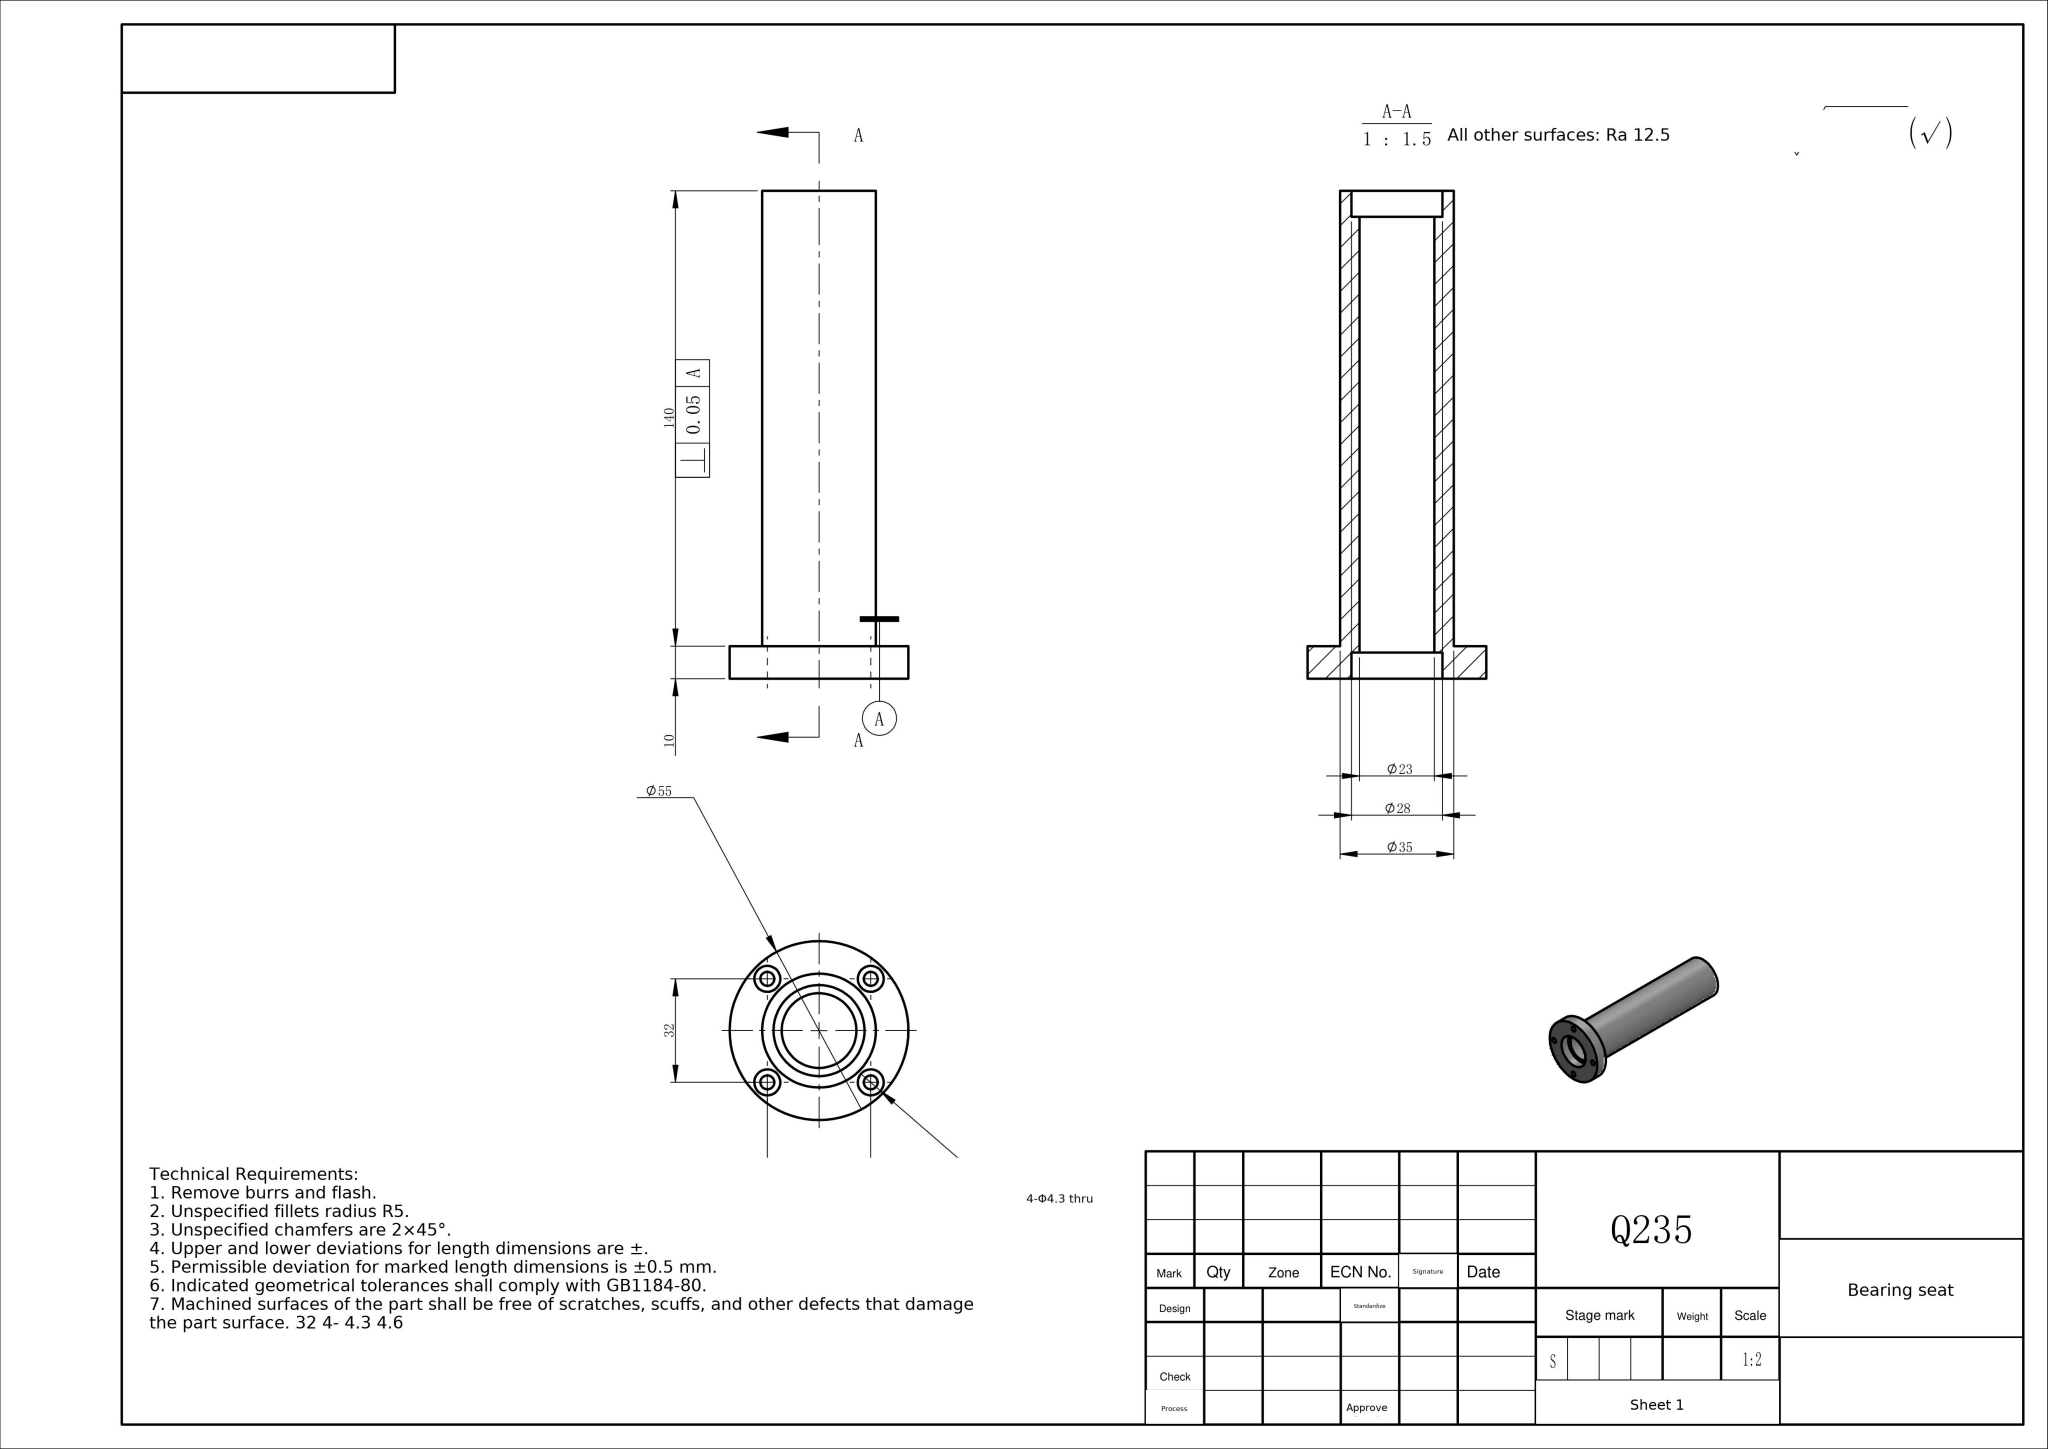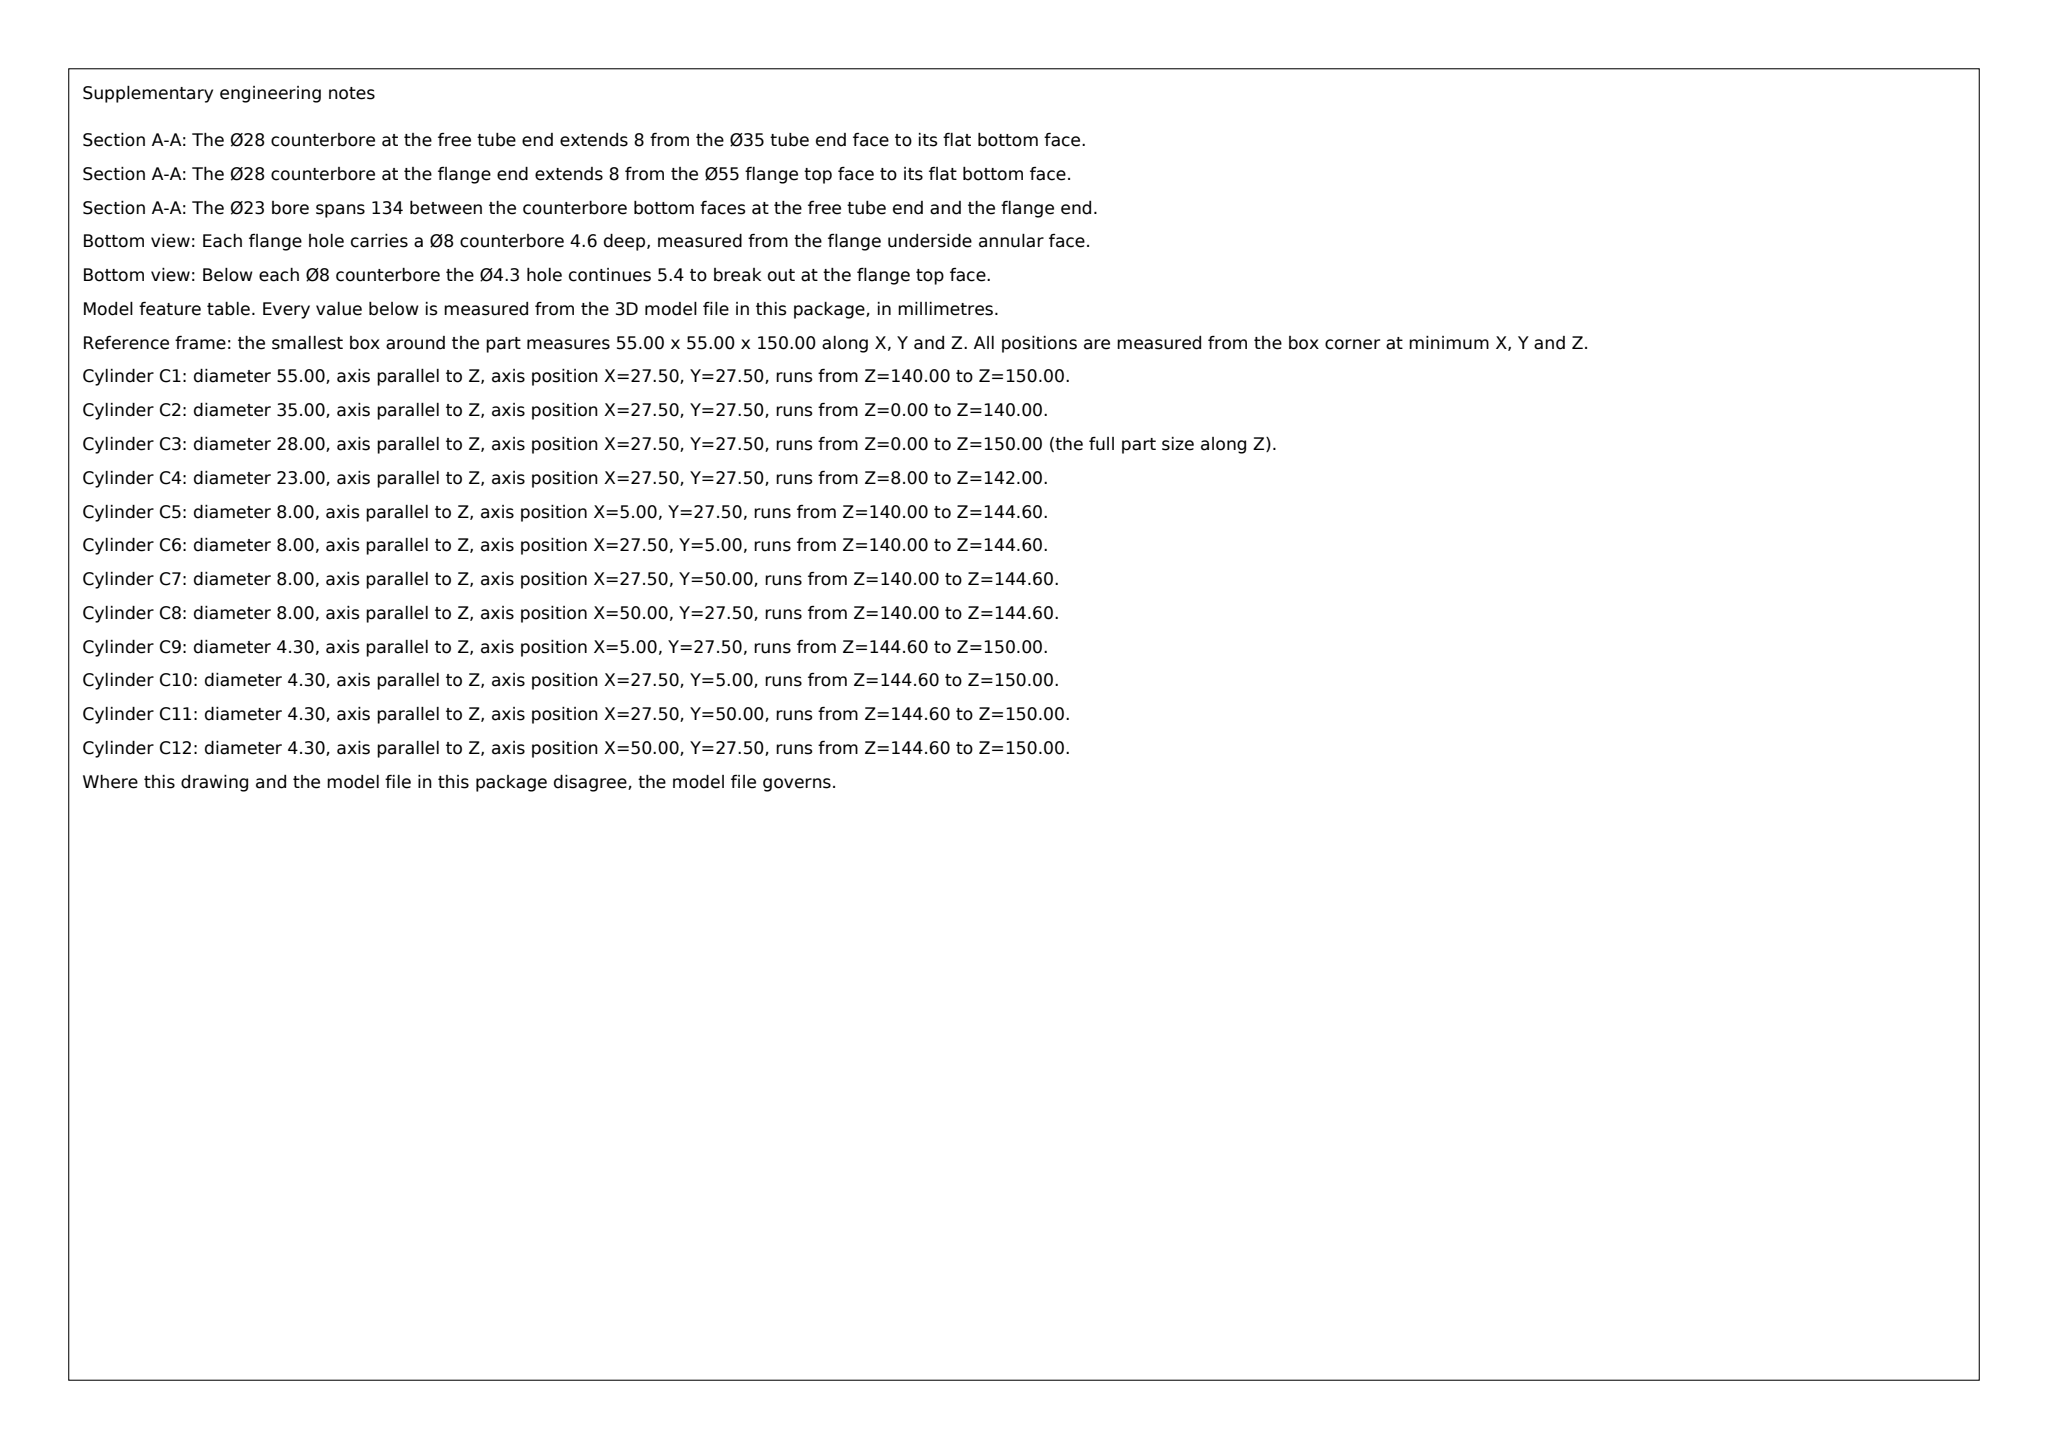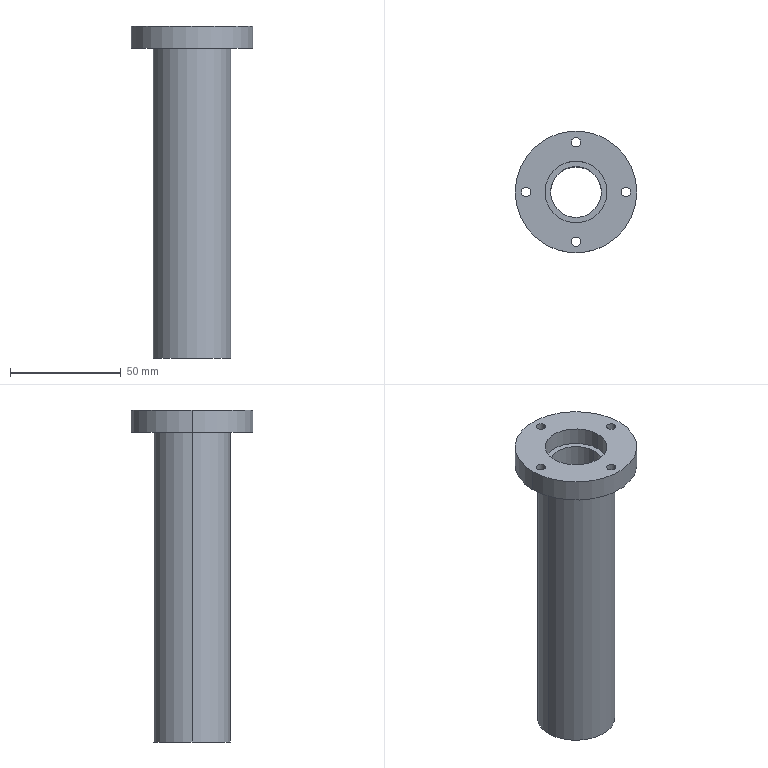Part | SolidWorks | mm | 1 solid | 35 faces | box 55 x 55 x 150 mm | volume 91690 mm3 | cylinder 26 | plane 9 | commonest cylinder face diameters 8 x8 4.3 x8 28 x4 23 x2 35 x2 55 x2
Drawing notes:
Ø28 COUNTERBORE 8 DEEP AT EACH END OF Ø23 BORE (both ends, concentric with Ø23); Ø23 BORE 134 LONG BETWEEN COUNTERBORES | from the solid: cylinders: [28,"z",[27.5,27.5],8.0] and [23,"z",[27.5,27.5],134.0]; axis planes z=8.0 and z=142.0
4X Ø4.3 HOLE PATTERN EQUALLY SPACED ON Ø45 BOLT CIRCLE, CENTRED ON THE TWO FLANGE CENTRE-LINES (0°/90°/180°/270°) | from the solid: cylinder positions [5.0,27.5],[27.5,5.0],[27.5,50.0],[50.0,27.5] vs part centre [27.5,27.5] → 22.5 radius on axes
4X Ø4.3 THRU, C'BORE Ø8 DEEP 4.6 FROM THE FLANGE FACE THAT MEETS THE Ø35 TUBE (Z=140); REMAINING Ø4.3 LENGTH 5.4 TO OUTER FLANGE FACE | from the solid: cylinders: [8.0,"z",4.6] and [4.3,"z",5.4]; axis_plane z=144.6 (count 4), flange faces z=140.0 and z=150.0